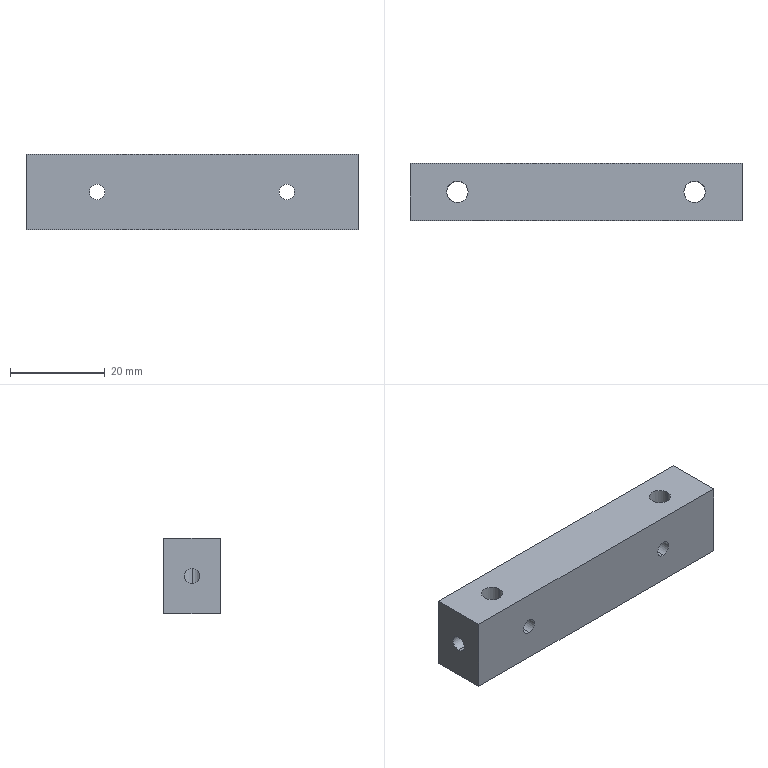Component | SolidWorks | InnerBagLiftingAluminumBlockA-1 | 1 solid | 18 faces | box 70 x 12 x 16 mm | volume 12590 mm3 | cylinder 12 | plane 6 | commonest cylinder face diameters 3.3 x8 4.5 x4
build123d program:
from build123d import *

# Parameters (mm, degrees)
SKETCH1_W             = 70
SKETCH1_H             = 12
BOSS_EXTRUDE1_DEPTH   = 8
SKETCH2_R             = 2.25
CUT_EXTRUDE1_DEPTH    = 73.801
M4_TAPPED_HOLE1_D     = 3.3
M4_TAPPED_HOLE2_D     = 3.3
M4_TAPPED_HOLE2_DEPTH = 10.1
M4_TAPPED_HOLE2_TIP   = 1.65
M4_TAPPED_HOLE3_D     = 3.3
M4_TAPPED_HOLE3_DEPTH = 10.1
M4_TAPPED_HOLE3_TIP   = 1.65


with BuildPart() as part:
    # Sketch1 → Boss-Extrude1 (new, symmetric)
    with BuildSketch(Plane.XY):
        with Locations((35, 6)):
            Rectangle(SKETCH1_W, SKETCH1_H)
    extrude(amount=BOSS_EXTRUDE1_DEPTH, both=True)

    # Sketch2 → Cut-Extrude1 (cut, through all)
    with BuildSketch(Plane.XY.offset(8)):
        with Locations((10, 6)):
            Circle(SKETCH2_R)
        with Locations((60, 6)):
            Circle(SKETCH2_R)
    extrude(amount=-CUT_EXTRUDE1_DEPTH, mode=Mode.SUBTRACT)

    # M4 Tapped Hole1 (through all)
    with Locations(Plane(origin=(15, 12, 0), x_dir=(0, 0, 1), z_dir=(0, 1, 0))):
        with Locations((0, 0), (0, 40)):
            Hole(M4_TAPPED_HOLE1_D / 2)

    # M4 Tapped Hole2
    with Locations(Plane(origin=(0, 6, 0), x_dir=(0, 0, -1), z_dir=(-1, 0, 0))):
        with Locations((0, 0)):
            Hole(M4_TAPPED_HOLE2_D / 2, depth=M4_TAPPED_HOLE2_DEPTH)
            with Locations((0, 0, -(M4_TAPPED_HOLE2_DEPTH + M4_TAPPED_HOLE2_TIP / 2))):  # 90° drill point
                Cone(0, M4_TAPPED_HOLE2_D / 2, M4_TAPPED_HOLE2_TIP, mode=Mode.SUBTRACT)

    # M4 Tapped Hole3
    with Locations(Plane(origin=(70, 6, 0), x_dir=(0, 0, 1), z_dir=(1, 0, 0))):
        with Locations((0, 0)):
            Hole(M4_TAPPED_HOLE3_D / 2, depth=M4_TAPPED_HOLE3_DEPTH)
            with Locations((0, 0, -(M4_TAPPED_HOLE3_DEPTH + M4_TAPPED_HOLE3_TIP / 2))):  # 90° drill point
                Cone(0, M4_TAPPED_HOLE3_D / 2, M4_TAPPED_HOLE3_TIP, mode=Mode.SUBTRACT)


solid = part.part

# Placed as in the assembly
solid = solid.moved(Location((29.354, -54.068, 156.933), (0, 0, 0)))
STEP:
#1=COLOUR_RGB('',0.7922,0.8196,0.9333);
#2=FILL_AREA_STYLE_COLOUR('',#1);
#3=FILL_AREA_STYLE('',(#2));
#4=SURFACE_STYLE_FILL_AREA(#3);
#5=SURFACE_SIDE_STYLE('',(#4));
#6=SURFACE_STYLE_USAGE(.BOTH.,#5);
#7=PRESENTATION_STYLE_ASSIGNMENT((#6));
#8=CARTESIAN_POINT('',(3.606,-1.892,6.243));
#9=VERTEX_POINT('',#8);
#10=CARTESIAN_POINT('',(3.606,-1.892,6.113));
#11=VERTEX_POINT('',#10);
#12=CARTESIAN_POINT('',(3.606,-1.892,6.243));
#13=CARTESIAN_POINT('',(3.606,-1.897,6.243));
#14=CARTESIAN_POINT('',(3.606,-1.901,6.243));
#15=CARTESIAN_POINT('',(3.605,-1.91,6.241));
#16=CARTESIAN_POINT('',(3.604,-1.914,6.24));
#17=CARTESIAN_POINT('',(3.6,-1.926,6.235));
#18=CARTESIAN_POINT('',(3.597,-1.933,6.23));
#19=CARTESIAN_POINT('',(3.59,-1.944,6.218));
#20=CARTESIAN_POINT('',(3.586,-1.949,6.211));
#21=CARTESIAN_POINT('',(3.58,-1.955,6.196));
#22=CARTESIAN_POINT('',(3.578,-1.957,6.187));
#23=CARTESIAN_POINT('',(3.578,-1.957,6.169));
#24=CARTESIAN_POINT('',(3.58,-1.955,6.161));
#25=CARTESIAN_POINT('',(3.585,-1.951,6.149));
#26=CARTESIAN_POINT('',(3.586,-1.949,6.146));
#27=CARTESIAN_POINT('',(3.59,-1.944,6.139));
#28=CARTESIAN_POINT('',(3.592,-1.941,6.136));
#29=CARTESIAN_POINT('',(3.595,-1.936,6.13));
#30=CARTESIAN_POINT('',(3.597,-1.933,6.127));
#31=CARTESIAN_POINT('',(3.6,-1.926,6.123));
#32=CARTESIAN_POINT('',(3.601,-1.922,6.12));
#33=CARTESIAN_POINT('',(3.605,-1.91,6.115));
#34=CARTESIAN_POINT('',(3.606,-1.901,6.113));
#35=CARTESIAN_POINT('',(3.606,-1.892,6.113));
#36=B_SPLINE_CURVE_WITH_KNOTS('',3,(#12,#13,#14,#15,#16,#17,#18,#19,#20,#21,#22,#23,#24,#25,#26,#27,#28,#29,#30,#31,#32,#33,#34,#35),.UNSPECIFIED.,.F.,.F.,(4,2,2,2,2,2,2,2,2,2,2,4),(0.005391,0.005727,0.006063,0.006736,0.007408,0.008081,0.008754,0.00909,0.009426,0.009762,0.0101,0.01077),.UNSPECIFIED.);
#37=EDGE_CURVE('',#9,#11,#36,.T.);
#38=ORIENTED_EDGE('',*,*,#37,.F.);
#39=CARTESIAN_POINT('',(3.912,-1.892,6.243));
#40=VERTEX_POINT('',#39);
#41=CARTESIAN_POINT('',(3.912,-1.892,6.243));
#42=DIRECTION('',(1.,0.,0.));
#43=VECTOR('',#42,39.37);
#44=LINE('',#41,#43);
#45=EDGE_CURVE('',#9,#40,#44,.T.);
#46=ORIENTED_EDGE('',*,*,#45,.T.);
#47=CARTESIAN_POINT('',(3.912,-1.892,6.113));
#48=VERTEX_POINT('',#47);
#49=CARTESIAN_POINT('',(3.912,-1.892,6.178));
#50=DIRECTION('',(1.,0.,0.));
#51=DIRECTION('',(0.,0.,-1.));
#52=AXIS2_PLACEMENT_3D('',#49,#50,#51);
#53=CIRCLE('',#52,0.06496);
#54=EDGE_CURVE('',#40,#48,#53,.T.);
#55=ORIENTED_EDGE('',*,*,#54,.T.);
#56=CARTESIAN_POINT('',(3.912,-1.892,6.113));
#57=DIRECTION('',(1.,0.,0.));
#58=VECTOR('',#57,39.37);
#59=LINE('',#56,#58);
#60=EDGE_CURVE('',#11,#48,#59,.T.);
#61=ORIENTED_EDGE('',*,*,#60,.F.);
#62=EDGE_LOOP('',(#38,#46,#55,#61));
#63=FACE_OUTER_BOUND('',#62,.T.);
#64=CARTESIAN_POINT('',(3.912,-1.892,6.178));
#65=DIRECTION('',(1.,0.,0.));
#66=DIRECTION('',(0.,0.,-1.));
#67=AXIS2_PLACEMENT_3D('',#64,#65,#66);
#68=CYLINDRICAL_SURFACE('',#67,0.06496);
#69=ADVANCED_FACE('',(#63),#68,.F.);
#70=CARTESIAN_POINT('',(1.461,-1.892,6.113));
#71=VERTEX_POINT('',#70);
#72=CARTESIAN_POINT('',(1.461,-1.892,6.243));
#73=VERTEX_POINT('',#72);
#74=CARTESIAN_POINT('',(1.461,-1.892,6.113));
#75=CARTESIAN_POINT('',(1.461,-1.897,6.113));
#76=CARTESIAN_POINT('',(1.461,-1.901,6.114));
#77=CARTESIAN_POINT('',(1.462,-1.91,6.116));
#78=CARTESIAN_POINT('',(1.463,-1.914,6.117));
#79=CARTESIAN_POINT('',(1.467,-1.926,6.122));
#80=CARTESIAN_POINT('',(1.47,-1.933,6.127));
#81=CARTESIAN_POINT('',(1.477,-1.944,6.139));
#82=CARTESIAN_POINT('',(1.481,-1.949,6.145));
#83=CARTESIAN_POINT('',(1.487,-1.955,6.161));
#84=CARTESIAN_POINT('',(1.489,-1.957,6.17));
#85=CARTESIAN_POINT('',(1.489,-1.957,6.187));
#86=CARTESIAN_POINT('',(1.487,-1.955,6.196));
#87=CARTESIAN_POINT('',(1.483,-1.951,6.208));
#88=CARTESIAN_POINT('',(1.481,-1.949,6.211));
#89=CARTESIAN_POINT('',(1.477,-1.944,6.218));
#90=CARTESIAN_POINT('',(1.476,-1.941,6.221));
#91=CARTESIAN_POINT('',(1.472,-1.936,6.227));
#92=CARTESIAN_POINT('',(1.47,-1.933,6.23));
#93=CARTESIAN_POINT('',(1.467,-1.926,6.234));
#94=CARTESIAN_POINT('',(1.466,-1.922,6.236));
#95=CARTESIAN_POINT('',(1.462,-1.91,6.242));
#96=CARTESIAN_POINT('',(1.461,-1.901,6.243));
#97=CARTESIAN_POINT('',(1.461,-1.892,6.243));
#98=B_SPLINE_CURVE_WITH_KNOTS('',3,(#74,#75,#76,#77,#78,#79,#80,#81,#82,#83,#84,#85,#86,#87,#88,#89,#90,#91,#92,#93,#94,#95,#96,#97),.UNSPECIFIED.,.F.,.F.,(4,2,2,2,2,2,2,2,2,2,2,4),(0.005391,0.005727,0.006063,0.006736,0.007408,0.008081,0.008754,0.00909,0.009426,0.009762,0.0101,0.01077),.UNSPECIFIED.);
#99=EDGE_CURVE('',#71,#73,#98,.T.);
#100=ORIENTED_EDGE('',*,*,#99,.F.);
#101=CARTESIAN_POINT('',(1.156,-1.892,6.113));
#102=VERTEX_POINT('',#101);
#103=CARTESIAN_POINT('',(1.156,-1.892,6.113));
#104=DIRECTION('',(-1.,0.,0.));
#105=VECTOR('',#104,39.37);
#106=LINE('',#103,#105);
#107=EDGE_CURVE('',#71,#102,#106,.T.);
#108=ORIENTED_EDGE('',*,*,#107,.T.);
#109=CARTESIAN_POINT('',(1.156,-1.892,6.243));
#110=VERTEX_POINT('',#109);
#111=CARTESIAN_POINT('',(1.156,-1.892,6.178));
#112=DIRECTION('',(-1.,0.,0.));
#113=DIRECTION('',(0.,0.,1.));
#114=AXIS2_PLACEMENT_3D('',#111,#112,#113);
#115=CIRCLE('',#114,0.06496);
#116=EDGE_CURVE('',#102,#110,#115,.T.);
#117=ORIENTED_EDGE('',*,*,#116,.T.);
#118=CARTESIAN_POINT('',(1.156,-1.892,6.243));
#119=DIRECTION('',(-1.,0.,0.));
#120=VECTOR('',#119,39.37);
#121=LINE('',#118,#120);
#122=EDGE_CURVE('',#73,#110,#121,.T.);
#123=ORIENTED_EDGE('',*,*,#122,.F.);
#124=EDGE_LOOP('',(#100,#108,#117,#123));
#125=FACE_OUTER_BOUND('',#124,.T.);
#126=CARTESIAN_POINT('',(1.156,-1.892,6.178));
#127=DIRECTION('',(-1.,0.,0.));
#128=DIRECTION('',(0.,0.,1.));
#129=AXIS2_PLACEMENT_3D('',#126,#127,#128);
#130=CYLINDRICAL_SURFACE('',#129,0.06496);
#131=ADVANCED_FACE('',(#125),#130,.F.);
#132=CARTESIAN_POINT('',(1.746,-2.129,6.113));
#133=VERTEX_POINT('',#132);
#134=CARTESIAN_POINT('',(1.746,-2.129,6.243));
#135=VERTEX_POINT('',#134);
#136=CARTESIAN_POINT('',(1.746,-2.129,6.178));
#137=DIRECTION('',(0.,1.,0.));
#138=DIRECTION('',(0.,0.,1.));
#139=AXIS2_PLACEMENT_3D('',#136,#137,#138);
#140=CIRCLE('',#139,0.06496);
#141=EDGE_CURVE('',#133,#135,#140,.T.);
#142=ORIENTED_EDGE('',*,*,#141,.F.);
#143=CARTESIAN_POINT('',(1.746,-1.656,6.113));
#144=VERTEX_POINT('',#143);
#145=CARTESIAN_POINT('',(1.746,-1.656,6.113));
#146=DIRECTION('',(0.,1.,0.));
#147=VECTOR('',#146,39.37);
#148=LINE('',#145,#147);
#149=EDGE_CURVE('',#133,#144,#148,.T.);
#150=ORIENTED_EDGE('',*,*,#149,.T.);
#151=CARTESIAN_POINT('',(1.746,-1.656,6.243));
#152=VERTEX_POINT('',#151);
#153=CARTESIAN_POINT('',(1.746,-1.656,6.178));
#154=DIRECTION('',(0.,1.,0.));
#155=DIRECTION('',(0.,0.,1.));
#156=AXIS2_PLACEMENT_3D('',#153,#154,#155);
#157=CIRCLE('',#156,0.06496);
#158=EDGE_CURVE('',#144,#152,#157,.T.);
#159=ORIENTED_EDGE('',*,*,#158,.T.);
#160=CARTESIAN_POINT('',(1.746,-1.656,6.243));
#161=DIRECTION('',(0.,1.,0.));
#162=VECTOR('',#161,39.37);
#163=LINE('',#160,#162);
#164=EDGE_CURVE('',#135,#152,#163,.T.);
#165=ORIENTED_EDGE('',*,*,#164,.F.);
#166=EDGE_LOOP('',(#142,#150,#159,#165));
#167=FACE_OUTER_BOUND('',#166,.T.);
#168=CARTESIAN_POINT('',(1.746,-1.656,6.178));
#169=DIRECTION('',(0.,1.,0.));
#170=DIRECTION('',(0.,0.,1.));
#171=AXIS2_PLACEMENT_3D('',#168,#169,#170);
#172=CYLINDRICAL_SURFACE('',#171,0.06496);
#173=ADVANCED_FACE('',(#167),#172,.F.);
#174=CARTESIAN_POINT('',(3.321,-2.129,6.113));
#175=VERTEX_POINT('',#174);
#176=CARTESIAN_POINT('',(3.321,-2.129,6.243));
#177=VERTEX_POINT('',#176);
#178=CARTESIAN_POINT('',(3.321,-2.129,6.178));
#179=DIRECTION('',(0.,1.,0.));
#180=DIRECTION('',(0.,0.,1.));
#181=AXIS2_PLACEMENT_3D('',#178,#179,#180);
#182=CIRCLE('',#181,0.06496);
#183=EDGE_CURVE('',#175,#177,#182,.T.);
#184=ORIENTED_EDGE('',*,*,#183,.F.);
#185=CARTESIAN_POINT('',(3.321,-1.656,6.113));
#186=VERTEX_POINT('',#185);
#187=CARTESIAN_POINT('',(3.321,-1.656,6.113));
#188=DIRECTION('',(0.,1.,0.));
#189=VECTOR('',#188,39.37);
#190=LINE('',#187,#189);
#191=EDGE_CURVE('',#175,#186,#190,.T.);
#192=ORIENTED_EDGE('',*,*,#191,.T.);
#193=CARTESIAN_POINT('',(3.321,-1.656,6.243));
#194=VERTEX_POINT('',#193);
#195=CARTESIAN_POINT('',(3.321,-1.656,6.178));
#196=DIRECTION('',(0.,1.,0.));
#197=DIRECTION('',(0.,0.,1.));
#198=AXIS2_PLACEMENT_3D('',#195,#196,#197);
#199=CIRCLE('',#198,0.06496);
#200=EDGE_CURVE('',#186,#194,#199,.T.);
#201=ORIENTED_EDGE('',*,*,#200,.T.);
#202=CARTESIAN_POINT('',(3.321,-1.656,6.243));
#203=DIRECTION('',(0.,1.,0.));
#204=VECTOR('',#203,39.37);
#205=LINE('',#202,#204);
#206=EDGE_CURVE('',#177,#194,#205,.T.);
#207=ORIENTED_EDGE('',*,*,#206,.F.);
#208=EDGE_LOOP('',(#184,#192,#201,#207));
#209=FACE_OUTER_BOUND('',#208,.T.);
#210=CARTESIAN_POINT('',(3.321,-1.656,6.178));
#211=DIRECTION('',(0.,1.,0.));
#212=DIRECTION('',(0.,0.,1.));
#213=AXIS2_PLACEMENT_3D('',#210,#211,#212);
#214=CYLINDRICAL_SURFACE('',#213,0.06496);
#215=ADVANCED_FACE('',(#209),#214,.F.);
#216=CARTESIAN_POINT('',(3.429,-1.892,5.863));
#217=VERTEX_POINT('',#216);
#218=CARTESIAN_POINT('',(3.606,-1.892,5.863));
#219=VERTEX_POINT('',#218);
#220=CARTESIAN_POINT('',(3.518,-1.892,5.863));
#221=DIRECTION('',(0.,0.,1.));
#222=DIRECTION('',(1.,0.,0.));
#223=AXIS2_PLACEMENT_3D('',#220,#221,#222);
#224=CIRCLE('',#223,0.08858);
#225=EDGE_CURVE('',#217,#219,#224,.T.);
#226=ORIENTED_EDGE('',*,*,#225,.F.);
#227=CARTESIAN_POINT('',(3.429,-1.892,6.493));
#228=VERTEX_POINT('',#227);
#229=CARTESIAN_POINT('',(3.429,-1.892,5.863));
#230=DIRECTION('',(0.,0.,1.));
#231=VECTOR('',#230,39.37);
#232=LINE('',#229,#231);
#233=EDGE_CURVE('',#217,#228,#232,.T.);
#234=ORIENTED_EDGE('',*,*,#233,.T.);
#235=CARTESIAN_POINT('',(3.606,-1.892,6.493));
#236=VERTEX_POINT('',#235);
#237=CARTESIAN_POINT('',(3.518,-1.892,6.493));
#238=DIRECTION('',(0.,0.,1.));
#239=DIRECTION('',(1.,0.,0.));
#240=AXIS2_PLACEMENT_3D('',#237,#238,#239);
#241=CIRCLE('',#240,0.08858);
#242=EDGE_CURVE('',#228,#236,#241,.T.);
#243=ORIENTED_EDGE('',*,*,#242,.T.);
#244=CARTESIAN_POINT('',(3.606,-1.892,5.863));
#245=DIRECTION('',(0.,0.,1.));
#246=VECTOR('',#245,39.37);
#247=LINE('',#244,#246);
#248=EDGE_CURVE('',#9,#236,#247,.T.);
#249=ORIENTED_EDGE('',*,*,#248,.F.);
#250=ORIENTED_EDGE('',*,*,#37,.T.);
#251=CARTESIAN_POINT('',(3.606,-1.892,5.863));
#252=DIRECTION('',(0.,0.,1.));
#253=VECTOR('',#252,39.37);
#254=LINE('',#251,#253);
#255=EDGE_CURVE('',#219,#11,#254,.T.);
#256=ORIENTED_EDGE('',*,*,#255,.F.);
#257=EDGE_LOOP('',(#226,#234,#243,#249,#250,#256));
#258=FACE_OUTER_BOUND('',#257,.T.);
#259=CARTESIAN_POINT('',(3.518,-1.892,5.863));
#260=DIRECTION('',(0.,0.,1.));
#261=DIRECTION('',(1.,0.,0.));
#262=AXIS2_PLACEMENT_3D('',#259,#260,#261);
#263=CYLINDRICAL_SURFACE('',#262,0.08858);
#264=ADVANCED_FACE('',(#258),#263,.F.);
#265=CARTESIAN_POINT('',(1.461,-1.892,5.863));
#266=VERTEX_POINT('',#265);
#267=CARTESIAN_POINT('',(1.638,-1.892,5.863));
#268=VERTEX_POINT('',#267);
#269=CARTESIAN_POINT('',(1.549,-1.892,5.863));
#270=DIRECTION('',(0.,0.,1.));
#271=DIRECTION('',(1.,0.,0.));
#272=AXIS2_PLACEMENT_3D('',#269,#270,#271);
#273=CIRCLE('',#272,0.08858);
#274=EDGE_CURVE('',#266,#268,#273,.T.);
#275=ORIENTED_EDGE('',*,*,#274,.F.);
#276=CARTESIAN_POINT('',(1.461,-1.892,5.863));
#277=DIRECTION('',(0.,0.,1.));
#278=VECTOR('',#277,39.37);
#279=LINE('',#276,#278);
#280=EDGE_CURVE('',#266,#71,#279,.T.);
#281=ORIENTED_EDGE('',*,*,#280,.T.);
#282=ORIENTED_EDGE('',*,*,#99,.T.);
#283=CARTESIAN_POINT('',(1.461,-1.892,6.493));
#284=VERTEX_POINT('',#283);
#285=CARTESIAN_POINT('',(1.461,-1.892,5.863));
#286=DIRECTION('',(0.,0.,1.));
#287=VECTOR('',#286,39.37);
#288=LINE('',#285,#287);
#289=EDGE_CURVE('',#73,#284,#288,.T.);
#290=ORIENTED_EDGE('',*,*,#289,.T.);
#291=CARTESIAN_POINT('',(1.638,-1.892,6.493));
#292=VERTEX_POINT('',#291);
#293=CARTESIAN_POINT('',(1.549,-1.892,6.493));
#294=DIRECTION('',(0.,0.,1.));
#295=DIRECTION('',(1.,0.,0.));
#296=AXIS2_PLACEMENT_3D('',#293,#294,#295);
#297=CIRCLE('',#296,0.08858);
#298=EDGE_CURVE('',#284,#292,#297,.T.);
#299=ORIENTED_EDGE('',*,*,#298,.T.);
#300=CARTESIAN_POINT('',(1.638,-1.892,5.863));
#301=DIRECTION('',(0.,0.,1.));
#302=VECTOR('',#301,39.37);
#303=LINE('',#300,#302);
#304=EDGE_CURVE('',#268,#292,#303,.T.);
#305=ORIENTED_EDGE('',*,*,#304,.F.);
#306=EDGE_LOOP('',(#275,#281,#282,#290,#299,#305));
#307=FACE_OUTER_BOUND('',#306,.T.);
#308=CARTESIAN_POINT('',(1.549,-1.892,5.863));
#309=DIRECTION('',(0.,0.,1.));
#310=DIRECTION('',(1.,0.,0.));
#311=AXIS2_PLACEMENT_3D('',#308,#309,#310);
#312=CYLINDRICAL_SURFACE('',#311,0.08858);
#313=ADVANCED_FACE('',(#307),#312,.F.);
#314=CARTESIAN_POINT('',(1.156,-1.892,6.178));
#315=DIRECTION('',(-1.,0.,0.));
#316=DIRECTION('',(0.,0.,1.));
#317=AXIS2_PLACEMENT_3D('',#314,#315,#316);
#318=CIRCLE('',#317,0.06496);
#319=EDGE_CURVE('',#110,#102,#318,.T.);
#320=ORIENTED_EDGE('',*,*,#319,.F.);
#321=ORIENTED_EDGE('',*,*,#116,.F.);
#322=EDGE_LOOP('',(#320,#321));
#323=FACE_BOUND('',#322,.T.);
#324=CARTESIAN_POINT('',(1.156,-1.656,5.863));
#325=VERTEX_POINT('',#324);
#326=CARTESIAN_POINT('',(1.156,-2.129,5.863));
#327=VERTEX_POINT('',#326);
#328=CARTESIAN_POINT('',(1.156,-2.129,5.863));
#329=DIRECTION('',(0.,-1.,0.));
#330=VECTOR('',#329,39.37);
#331=LINE('',#328,#330);
#332=EDGE_CURVE('',#325,#327,#331,.T.);
#333=ORIENTED_EDGE('',*,*,#332,.T.);
#334=CARTESIAN_POINT('',(1.156,-2.129,6.493));
#335=VERTEX_POINT('',#334);
#336=CARTESIAN_POINT('',(1.156,-2.129,6.493));
#337=DIRECTION('',(0.,0.,-1.));
#338=VECTOR('',#337,39.37);
#339=LINE('',#336,#338);
#340=EDGE_CURVE('',#335,#327,#339,.T.);
#341=ORIENTED_EDGE('',*,*,#340,.F.);
#342=CARTESIAN_POINT('',(1.156,-1.656,6.493));
#343=VERTEX_POINT('',#342);
#344=CARTESIAN_POINT('',(1.156,-2.129,6.493));
#345=DIRECTION('',(0.,-1.,0.));
#346=VECTOR('',#345,39.37);
#347=LINE('',#344,#346);
#348=EDGE_CURVE('',#343,#335,#347,.T.);
#349=ORIENTED_EDGE('',*,*,#348,.F.);
#350=CARTESIAN_POINT('',(1.156,-1.656,6.493));
#351=DIRECTION('',(0.,0.,-1.));
#352=VECTOR('',#351,39.37);
#353=LINE('',#350,#352);
#354=EDGE_CURVE('',#343,#325,#353,.T.);
#355=ORIENTED_EDGE('',*,*,#354,.T.);
#356=EDGE_LOOP('',(#333,#341,#349,#355));
#357=FACE_OUTER_BOUND('',#356,.T.);
#358=CARTESIAN_POINT('',(1.156,-2.129,6.493));
#359=DIRECTION('',(1.,0.,0.));
#360=DIRECTION('',(0.,0.,-1.));
#361=AXIS2_PLACEMENT_3D('',#358,#359,#360);
#362=PLANE('',#361);
#363=ADVANCED_FACE('',(#323,#357),#362,.F.);
#364=CARTESIAN_POINT('',(1.746,-2.129,6.178));
#365=DIRECTION('',(0.,1.,0.));
#366=DIRECTION('',(0.,0.,1.));
#367=AXIS2_PLACEMENT_3D('',#364,#365,#366);
#368=CIRCLE('',#367,0.06496);
#369=EDGE_CURVE('',#135,#133,#368,.T.);
#370=ORIENTED_EDGE('',*,*,#369,.T.);
#371=ORIENTED_EDGE('',*,*,#141,.T.);
#372=EDGE_LOOP('',(#370,#371));
#373=FACE_BOUND('',#372,.T.);
#374=CARTESIAN_POINT('',(3.321,-2.129,6.178));
#375=DIRECTION('',(0.,1.,0.));
#376=DIRECTION('',(0.,0.,1.));
#377=AXIS2_PLACEMENT_3D('',#374,#375,#376);
#378=CIRCLE('',#377,0.06496);
#379=EDGE_CURVE('',#177,#175,#378,.T.);
#380=ORIENTED_EDGE('',*,*,#379,.T.);
#381=ORIENTED_EDGE('',*,*,#183,.T.);
#382=EDGE_LOOP('',(#380,#381));
#383=FACE_BOUND('',#382,.T.);
#384=CARTESIAN_POINT('',(3.912,-2.129,5.863));
#385=VERTEX_POINT('',#384);
#386=CARTESIAN_POINT('',(1.156,-2.129,5.863));
#387=DIRECTION('',(1.,0.,0.));
#388=VECTOR('',#387,39.37);
#389=LINE('',#386,#388);
#390=EDGE_CURVE('',#327,#385,#389,.T.);
#391=ORIENTED_EDGE('',*,*,#390,.T.);
#392=CARTESIAN_POINT('',(3.912,-2.129,6.493));
#393=VERTEX_POINT('',#392);
#394=CARTESIAN_POINT('',(3.912,-2.129,6.493));
#395=DIRECTION('',(0.,0.,-1.));
#396=VECTOR('',#395,39.37);
#397=LINE('',#394,#396);
#398=EDGE_CURVE('',#393,#385,#397,.T.);
#399=ORIENTED_EDGE('',*,*,#398,.F.);
#400=CARTESIAN_POINT('',(1.156,-2.129,6.493));
#401=DIRECTION('',(1.,0.,0.));
#402=VECTOR('',#401,39.37);
#403=LINE('',#400,#402);
#404=EDGE_CURVE('',#335,#393,#403,.T.);
#405=ORIENTED_EDGE('',*,*,#404,.F.);
#406=ORIENTED_EDGE('',*,*,#340,.T.);
#407=EDGE_LOOP('',(#391,#399,#405,#406));
#408=FACE_OUTER_BOUND('',#407,.T.);
#409=CARTESIAN_POINT('',(1.156,-2.129,6.493));
#410=DIRECTION('',(0.,1.,0.));
#411=DIRECTION('',(0.,0.,1.));
#412=AXIS2_PLACEMENT_3D('',#409,#410,#411);
#413=PLANE('',#412);
#414=ADVANCED_FACE('',(#373,#383,#408),#413,.F.);
#415=CARTESIAN_POINT('',(3.912,-1.892,6.178));
#416=DIRECTION('',(1.,0.,0.));
#417=DIRECTION('',(0.,0.,-1.));
#418=AXIS2_PLACEMENT_3D('',#415,#416,#417);
#419=CIRCLE('',#418,0.06496);
#420=EDGE_CURVE('',#48,#40,#419,.T.);
#421=ORIENTED_EDGE('',*,*,#420,.F.);
#422=ORIENTED_EDGE('',*,*,#54,.F.);
#423=EDGE_LOOP('',(#421,#422));
#424=FACE_BOUND('',#423,.T.);
#425=CARTESIAN_POINT('',(3.912,-1.656,5.863));
#426=VERTEX_POINT('',#425);
#427=CARTESIAN_POINT('',(3.912,-2.129,5.863));
#428=DIRECTION('',(0.,1.,0.));
#429=VECTOR('',#428,39.37);
#430=LINE('',#427,#429);
#431=EDGE_CURVE('',#385,#426,#430,.T.);
#432=ORIENTED_EDGE('',*,*,#431,.T.);
#433=CARTESIAN_POINT('',(3.912,-1.656,6.493));
#434=VERTEX_POINT('',#433);
#435=CARTESIAN_POINT('',(3.912,-1.656,6.493));
#436=DIRECTION('',(0.,0.,-1.));
#437=VECTOR('',#436,39.37);
#438=LINE('',#435,#437);
#439=EDGE_CURVE('',#434,#426,#438,.T.);
#440=ORIENTED_EDGE('',*,*,#439,.F.);
#441=CARTESIAN_POINT('',(3.912,-2.129,6.493));
#442=DIRECTION('',(0.,1.,0.));
#443=VECTOR('',#442,39.37);
#444=LINE('',#441,#443);
#445=EDGE_CURVE('',#393,#434,#444,.T.);
#446=ORIENTED_EDGE('',*,*,#445,.F.);
#447=ORIENTED_EDGE('',*,*,#398,.T.);
#448=EDGE_LOOP('',(#432,#440,#446,#447));
#449=FACE_OUTER_BOUND('',#448,.T.);
#450=CARTESIAN_POINT('',(3.912,-2.129,6.493));
#451=DIRECTION('',(-1.,0.,0.));
#452=DIRECTION('',(0.,0.,1.));
#453=AXIS2_PLACEMENT_3D('',#450,#451,#452);
#454=PLANE('',#453);
#455=ADVANCED_FACE('',(#424,#449),#454,.F.);
#456=CARTESIAN_POINT('',(1.746,-1.656,6.178));
#457=DIRECTION('',(0.,1.,0.));
#458=DIRECTION('',(0.,0.,1.));
#459=AXIS2_PLACEMENT_3D('',#456,#457,#458);
#460=CIRCLE('',#459,0.06496);
#461=EDGE_CURVE('',#152,#144,#460,.T.);
#462=ORIENTED_EDGE('',*,*,#461,.F.);
#463=ORIENTED_EDGE('',*,*,#158,.F.);
#464=EDGE_LOOP('',(#462,#463));
#465=FACE_BOUND('',#464,.T.);
#466=CARTESIAN_POINT('',(3.321,-1.656,6.178));
#467=DIRECTION('',(0.,1.,0.));
#468=DIRECTION('',(0.,0.,1.));
#469=AXIS2_PLACEMENT_3D('',#466,#467,#468);
#470=CIRCLE('',#469,0.06496);
#471=EDGE_CURVE('',#194,#186,#470,.T.);
#472=ORIENTED_EDGE('',*,*,#471,.F.);
#473=ORIENTED_EDGE('',*,*,#200,.F.);
#474=EDGE_LOOP('',(#472,#473));
#475=FACE_BOUND('',#474,.T.);
#476=CARTESIAN_POINT('',(1.156,-1.656,5.863));
#477=DIRECTION('',(-1.,0.,0.));
#478=VECTOR('',#477,39.37);
#479=LINE('',#476,#478);
#480=EDGE_CURVE('',#426,#325,#479,.T.);
#481=ORIENTED_EDGE('',*,*,#480,.T.);
#482=ORIENTED_EDGE('',*,*,#354,.F.);
#483=CARTESIAN_POINT('',(1.156,-1.656,6.493));
#484=DIRECTION('',(-1.,0.,0.));
#485=VECTOR('',#484,39.37);
#486=LINE('',#483,#485);
#487=EDGE_CURVE('',#434,#343,#486,.T.);
#488=ORIENTED_EDGE('',*,*,#487,.F.);
#489=ORIENTED_EDGE('',*,*,#439,.T.);
#490=EDGE_LOOP('',(#481,#482,#488,#489));
#491=FACE_OUTER_BOUND('',#490,.T.);
#492=CARTESIAN_POINT('',(1.156,-1.656,6.493));
#493=DIRECTION('',(0.,-1.,0.));
#494=DIRECTION('',(0.,0.,-1.));
#495=AXIS2_PLACEMENT_3D('',#492,#493,#494);
#496=PLANE('',#495);
#497=ADVANCED_FACE('',(#465,#475,#491),#496,.F.);
#498=CARTESIAN_POINT('',(3.518,-1.892,6.493));
#499=DIRECTION('',(0.,0.,1.));
#500=DIRECTION('',(1.,0.,0.));
#501=AXIS2_PLACEMENT_3D('',#498,#499,#500);
#502=CIRCLE('',#501,0.08858);
#503=EDGE_CURVE('',#236,#228,#502,.T.);
#504=ORIENTED_EDGE('',*,*,#503,.F.);
#505=ORIENTED_EDGE('',*,*,#242,.F.);
#506=EDGE_LOOP('',(#504,#505));
#507=FACE_BOUND('',#506,.T.);
#508=CARTESIAN_POINT('',(1.549,-1.892,6.493));
#509=DIRECTION('',(0.,0.,1.));
#510=DIRECTION('',(1.,0.,0.));
#511=AXIS2_PLACEMENT_3D('',#508,#509,#510);
#512=CIRCLE('',#511,0.08858);
#513=EDGE_CURVE('',#292,#284,#512,.T.);
#514=ORIENTED_EDGE('',*,*,#513,.F.);
#515=ORIENTED_EDGE('',*,*,#298,.F.);
#516=EDGE_LOOP('',(#514,#515));
#517=FACE_BOUND('',#516,.T.);
#518=ORIENTED_EDGE('',*,*,#348,.T.);
#519=ORIENTED_EDGE('',*,*,#404,.T.);
#520=ORIENTED_EDGE('',*,*,#445,.T.);
#521=ORIENTED_EDGE('',*,*,#487,.T.);
#522=EDGE_LOOP('',(#518,#519,#520,#521));
#523=FACE_OUTER_BOUND('',#522,.T.);
#524=CARTESIAN_POINT('',(1.156,-2.129,6.493));
#525=DIRECTION('',(0.,0.,-1.));
#526=DIRECTION('',(-1.,0.,0.));
#527=AXIS2_PLACEMENT_3D('',#524,#525,#526);
#528=PLANE('',#527);
#529=ADVANCED_FACE('',(#507,#517,#523),#528,.F.);
#530=CARTESIAN_POINT('',(3.518,-1.892,5.863));
#531=DIRECTION('',(0.,0.,1.));
#532=DIRECTION('',(1.,0.,0.));
#533=AXIS2_PLACEMENT_3D('',#530,#531,#532);
#534=CIRCLE('',#533,0.08858);
#535=EDGE_CURVE('',#219,#217,#534,.T.);
#536=ORIENTED_EDGE('',*,*,#535,.T.);
#537=ORIENTED_EDGE('',*,*,#225,.T.);
#538=EDGE_LOOP('',(#536,#537));
#539=FACE_BOUND('',#538,.T.);
#540=CARTESIAN_POINT('',(1.549,-1.892,5.863));
#541=DIRECTION('',(0.,0.,1.));
#542=DIRECTION('',(1.,0.,0.));
#543=AXIS2_PLACEMENT_3D('',#540,#541,#542);
#544=CIRCLE('',#543,0.08858);
#545=EDGE_CURVE('',#268,#266,#544,.T.);
#546=ORIENTED_EDGE('',*,*,#545,.T.);
#547=ORIENTED_EDGE('',*,*,#274,.T.);
#548=EDGE_LOOP('',(#546,#547));
#549=FACE_BOUND('',#548,.T.);
#550=ORIENTED_EDGE('',*,*,#332,.F.);
#551=ORIENTED_EDGE('',*,*,#480,.F.);
#552=ORIENTED_EDGE('',*,*,#431,.F.);
#553=ORIENTED_EDGE('',*,*,#390,.F.);
#554=EDGE_LOOP('',(#550,#551,#552,#553));
#555=FACE_OUTER_BOUND('',#554,.T.);
#556=CARTESIAN_POINT('',(1.156,-2.129,5.863));
#557=DIRECTION('',(0.,0.,-1.));
#558=DIRECTION('',(-1.,0.,0.));
#559=AXIS2_PLACEMENT_3D('',#556,#557,#558);
#560=PLANE('',#559);
#561=ADVANCED_FACE('',(#539,#549,#555),#560,.T.);
#562=ORIENTED_EDGE('',*,*,#280,.F.);
#563=ORIENTED_EDGE('',*,*,#545,.F.);
#564=ORIENTED_EDGE('',*,*,#304,.T.);
#565=ORIENTED_EDGE('',*,*,#513,.T.);
#566=ORIENTED_EDGE('',*,*,#289,.F.);
#567=CARTESIAN_POINT('',(1.461,-1.892,6.243));
#568=CARTESIAN_POINT('',(1.461,-1.888,6.243));
#569=CARTESIAN_POINT('',(1.461,-1.884,6.243));
#570=CARTESIAN_POINT('',(1.462,-1.875,6.241));
#571=CARTESIAN_POINT('',(1.463,-1.871,6.24));
#572=CARTESIAN_POINT('',(1.467,-1.859,6.235));
#573=CARTESIAN_POINT('',(1.47,-1.852,6.23));
#574=CARTESIAN_POINT('',(1.476,-1.843,6.221));
#575=CARTESIAN_POINT('',(1.477,-1.841,6.218));
#576=CARTESIAN_POINT('',(1.481,-1.836,6.211));
#577=CARTESIAN_POINT('',(1.483,-1.834,6.208));
#578=CARTESIAN_POINT('',(1.486,-1.831,6.2));
#579=CARTESIAN_POINT('',(1.487,-1.83,6.196));
#580=CARTESIAN_POINT('',(1.489,-1.828,6.187));
#581=CARTESIAN_POINT('',(1.489,-1.827,6.183));
#582=CARTESIAN_POINT('',(1.489,-1.827,6.174));
#583=CARTESIAN_POINT('',(1.489,-1.828,6.17));
#584=CARTESIAN_POINT('',(1.487,-1.83,6.161));
#585=CARTESIAN_POINT('',(1.486,-1.831,6.157));
#586=CARTESIAN_POINT('',(1.481,-1.836,6.145));
#587=CARTESIAN_POINT('',(1.477,-1.84,6.139));
#588=CARTESIAN_POINT('',(1.47,-1.852,6.127));
#589=CARTESIAN_POINT('',(1.467,-1.859,6.122));
#590=CARTESIAN_POINT('',(1.463,-1.871,6.117));
#591=CARTESIAN_POINT('',(1.462,-1.875,6.116));
#592=CARTESIAN_POINT('',(1.461,-1.883,6.114));
#593=CARTESIAN_POINT('',(1.461,-1.888,6.113));
#594=CARTESIAN_POINT('',(1.461,-1.892,6.113));
#595=B_SPLINE_CURVE_WITH_KNOTS('',3,(#567,#568,#569,#570,#571,#572,#573,#574,#575,#576,#577,#578,#579,#580,#581,#582,#583,#584,#585,#586,#587,#588,#589,#590,#591,#592,#593,#594),.UNSPECIFIED.,.F.,.F.,(4,2,2,2,2,2,2,2,2,2,2,2,2,4),(0.,0.0003369,0.0006738,0.001348,0.001685,0.002022,0.002358,0.002695,0.003032,0.003369,0.004043,0.004717,0.005054,0.005391),.UNSPECIFIED.);
#596=EDGE_CURVE('',#73,#71,#595,.T.);
#597=ORIENTED_EDGE('',*,*,#596,.T.);
#598=EDGE_LOOP('',(#562,#563,#564,#565,#566,#597));
#599=FACE_OUTER_BOUND('',#598,.T.);
#600=CARTESIAN_POINT('',(1.549,-1.892,5.863));
#601=DIRECTION('',(0.,0.,1.));
#602=DIRECTION('',(1.,0.,0.));
#603=AXIS2_PLACEMENT_3D('',#600,#601,#602);
#604=CYLINDRICAL_SURFACE('',#603,0.08858);
#605=ADVANCED_FACE('',(#599),#604,.F.);
#606=ORIENTED_EDGE('',*,*,#233,.F.);
#607=ORIENTED_EDGE('',*,*,#535,.F.);
#608=ORIENTED_EDGE('',*,*,#255,.T.);
#609=CARTESIAN_POINT('',(3.606,-1.892,6.113));
#610=CARTESIAN_POINT('',(3.606,-1.888,6.113));
#611=CARTESIAN_POINT('',(3.606,-1.884,6.114));
#612=CARTESIAN_POINT('',(3.605,-1.875,6.116));
#613=CARTESIAN_POINT('',(3.604,-1.871,6.117));
#614=CARTESIAN_POINT('',(3.6,-1.859,6.122));
#615=CARTESIAN_POINT('',(3.597,-1.852,6.127));
#616=CARTESIAN_POINT('',(3.592,-1.843,6.136));
#617=CARTESIAN_POINT('',(3.59,-1.841,6.139));
#618=CARTESIAN_POINT('',(3.586,-1.836,6.146));
#619=CARTESIAN_POINT('',(3.585,-1.834,6.149));
#620=CARTESIAN_POINT('',(3.582,-1.831,6.157));
#621=CARTESIAN_POINT('',(3.58,-1.83,6.161));
#622=CARTESIAN_POINT('',(3.579,-1.828,6.17));
#623=CARTESIAN_POINT('',(3.578,-1.827,6.174));
#624=CARTESIAN_POINT('',(3.578,-1.827,6.183));
#625=CARTESIAN_POINT('',(3.579,-1.828,6.187));
#626=CARTESIAN_POINT('',(3.58,-1.83,6.196));
#627=CARTESIAN_POINT('',(3.582,-1.831,6.2));
#628=CARTESIAN_POINT('',(3.586,-1.836,6.212));
#629=CARTESIAN_POINT('',(3.59,-1.84,6.218));
#630=CARTESIAN_POINT('',(3.597,-1.852,6.23));
#631=CARTESIAN_POINT('',(3.6,-1.859,6.235));
#632=CARTESIAN_POINT('',(3.604,-1.871,6.24));
#633=CARTESIAN_POINT('',(3.605,-1.875,6.241));
#634=CARTESIAN_POINT('',(3.606,-1.883,6.243));
#635=CARTESIAN_POINT('',(3.606,-1.888,6.243));
#636=CARTESIAN_POINT('',(3.606,-1.892,6.243));
#637=B_SPLINE_CURVE_WITH_KNOTS('',3,(#609,#610,#611,#612,#613,#614,#615,#616,#617,#618,#619,#620,#621,#622,#623,#624,#625,#626,#627,#628,#629,#630,#631,#632,#633,#634,#635,#636),.UNSPECIFIED.,.F.,.F.,(4,2,2,2,2,2,2,2,2,2,2,2,2,4),(0.,0.0003369,0.0006738,0.001348,0.001685,0.002022,0.002358,0.002695,0.003032,0.003369,0.004043,0.004717,0.005054,0.005391),.UNSPECIFIED.);
#638=EDGE_CURVE('',#11,#9,#637,.T.);
#639=ORIENTED_EDGE('',*,*,#638,.T.);
#640=ORIENTED_EDGE('',*,*,#248,.T.);
#641=ORIENTED_EDGE('',*,*,#503,.T.);
#642=EDGE_LOOP('',(#606,#607,#608,#639,#640,#641));
#643=FACE_OUTER_BOUND('',#642,.T.);
#644=CARTESIAN_POINT('',(3.518,-1.892,5.863));
#645=DIRECTION('',(0.,0.,1.));
#646=DIRECTION('',(1.,0.,0.));
#647=AXIS2_PLACEMENT_3D('',#644,#645,#646);
#648=CYLINDRICAL_SURFACE('',#647,0.08858);
#649=ADVANCED_FACE('',(#643),#648,.F.);
#650=ORIENTED_EDGE('',*,*,#191,.F.);
#651=ORIENTED_EDGE('',*,*,#379,.F.);
#652=ORIENTED_EDGE('',*,*,#206,.T.);
#653=ORIENTED_EDGE('',*,*,#471,.T.);
#654=EDGE_LOOP('',(#650,#651,#652,#653));
#655=FACE_OUTER_BOUND('',#654,.T.);
#656=CARTESIAN_POINT('',(3.321,-1.656,6.178));
#657=DIRECTION('',(0.,1.,0.));
#658=DIRECTION('',(0.,0.,1.));
#659=AXIS2_PLACEMENT_3D('',#656,#657,#658);
#660=CYLINDRICAL_SURFACE('',#659,0.06496);
#661=ADVANCED_FACE('',(#655),#660,.F.);
#662=ORIENTED_EDGE('',*,*,#149,.F.);
#663=ORIENTED_EDGE('',*,*,#369,.F.);
#664=ORIENTED_EDGE('',*,*,#164,.T.);
#665=ORIENTED_EDGE('',*,*,#461,.T.);
#666=EDGE_LOOP('',(#662,#663,#664,#665));
#667=FACE_OUTER_BOUND('',#666,.T.);
#668=CARTESIAN_POINT('',(1.746,-1.656,6.178));
#669=DIRECTION('',(0.,1.,0.));
#670=DIRECTION('',(0.,0.,1.));
#671=AXIS2_PLACEMENT_3D('',#668,#669,#670);
#672=CYLINDRICAL_SURFACE('',#671,0.06496);
#673=ADVANCED_FACE('',(#667),#672,.F.);
#674=ORIENTED_EDGE('',*,*,#107,.F.);
#675=ORIENTED_EDGE('',*,*,#596,.F.);
#676=ORIENTED_EDGE('',*,*,#122,.T.);
#677=ORIENTED_EDGE('',*,*,#319,.T.);
#678=EDGE_LOOP('',(#674,#675,#676,#677));
#679=FACE_OUTER_BOUND('',#678,.T.);
#680=CARTESIAN_POINT('',(1.156,-1.892,6.178));
#681=DIRECTION('',(-1.,0.,0.));
#682=DIRECTION('',(0.,0.,1.));
#683=AXIS2_PLACEMENT_3D('',#680,#681,#682);
#684=CYLINDRICAL_SURFACE('',#683,0.06496);
#685=ADVANCED_FACE('',(#679),#684,.F.);
#686=ORIENTED_EDGE('',*,*,#45,.F.);
#687=ORIENTED_EDGE('',*,*,#638,.F.);
#688=ORIENTED_EDGE('',*,*,#60,.T.);
#689=ORIENTED_EDGE('',*,*,#420,.T.);
#690=EDGE_LOOP('',(#686,#687,#688,#689));
#691=FACE_OUTER_BOUND('',#690,.T.);
#692=CARTESIAN_POINT('',(3.912,-1.892,6.178));
#693=DIRECTION('',(1.,0.,0.));
#694=DIRECTION('',(0.,0.,-1.));
#695=AXIS2_PLACEMENT_3D('',#692,#693,#694);
#696=CYLINDRICAL_SURFACE('',#695,0.06496);
#697=ADVANCED_FACE('',(#691),#696,.F.);
#698=CLOSED_SHELL('',(#69,#131,#173,#215,#264,#313,#363,#414,#455,#497,#529,#561,#605,#649,#661,#673,#685,#697));
#699=MANIFOLD_SOLID_BREP('',#698);
#700=STYLED_ITEM('',(#7),#699);
#701=PRESENTATION_LAYER_ASSIGNMENT('','',(#700));
#702=(LENGTH_UNIT()NAMED_UNIT(*)SI_UNIT($,.METRE.));
#703=LENGTH_MEASURE_WITH_UNIT(LENGTH_MEASURE(0.0254),#702);
#704=DIMENSIONAL_EXPONENTS(1.,0.,0.,0.,0.,0.,0.);
#705=(CONVERSION_BASED_UNIT('',#703)LENGTH_UNIT()NAMED_UNIT(#704));
#706=UNCERTAINTY_MEASURE_WITH_UNIT(LENGTH_MEASURE(0.00001),#705,'','');
#707=(NAMED_UNIT(*)PLANE_ANGLE_UNIT()SI_UNIT($,.RADIAN.));
#708=(NAMED_UNIT(*)SI_UNIT($,.STERADIAN.)SOLID_ANGLE_UNIT());
#709=(GEOMETRIC_REPRESENTATION_CONTEXT(3)GLOBAL_UNCERTAINTY_ASSIGNED_CONTEXT((#706))GLOBAL_UNIT_ASSIGNED_CONTEXT((#705,#707,#708))REPRESENTATION_CONTEXT('',''));
#710=MECHANICAL_DESIGN_GEOMETRIC_PRESENTATION_REPRESENTATION('',(#700),#709);
#711=CARTESIAN_POINT('',(0.,0.,0.));
#712=DIRECTION('',(0.,0.,1.));
#713=DIRECTION('',(1.,0.,0.));
#714=AXIS2_PLACEMENT_3D('',#711,#712,#713);
#715=(LENGTH_UNIT()NAMED_UNIT(*)SI_UNIT($,.METRE.));
#716=LENGTH_MEASURE_WITH_UNIT(LENGTH_MEASURE(0.0254),#715);
#717=DIMENSIONAL_EXPONENTS(1.,0.,0.,0.,0.,0.,0.);
#718=(CONVERSION_BASED_UNIT('',#716)LENGTH_UNIT()NAMED_UNIT(#717));
#719=UNCERTAINTY_MEASURE_WITH_UNIT(LENGTH_MEASURE(0.00001),#718,'','');
#720=(NAMED_UNIT(*)PLANE_ANGLE_UNIT()SI_UNIT($,.RADIAN.));
#721=(NAMED_UNIT(*)SI_UNIT($,.STERADIAN.)SOLID_ANGLE_UNIT());
#722=(GEOMETRIC_REPRESENTATION_CONTEXT(3)GLOBAL_UNCERTAINTY_ASSIGNED_CONTEXT((#719))GLOBAL_UNIT_ASSIGNED_CONTEXT((#718,#720,#721))REPRESENTATION_CONTEXT('',''));
#723=ADVANCED_BREP_SHAPE_REPRESENTATION('',(#699,#714),#722);